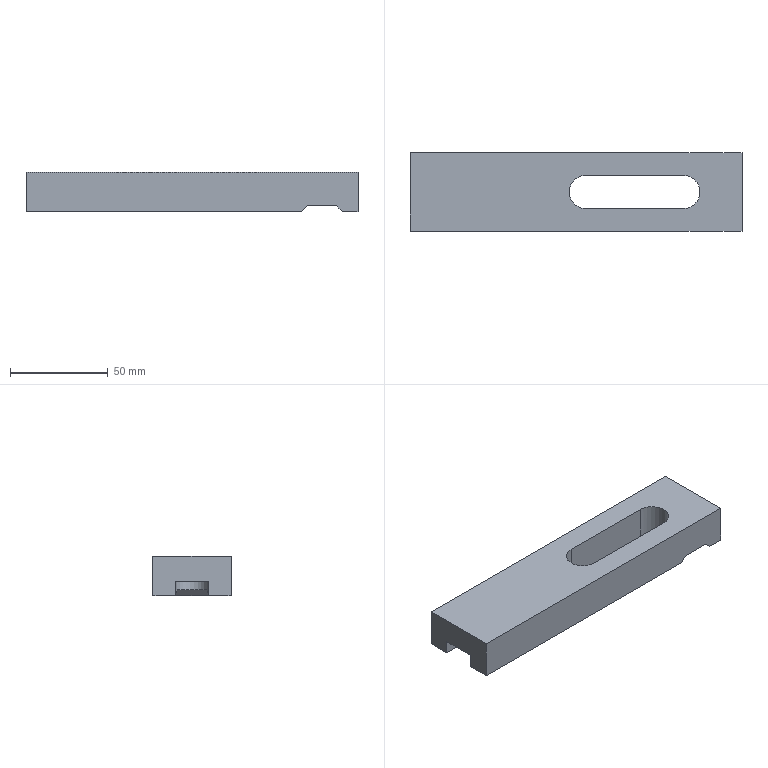Component | NX | CLAMP_PLATE | 1 solid | 17 faces | volume 102600 mm3 | plane 15 | cylinder 2 | commonest cylinder face diameters 17 x2